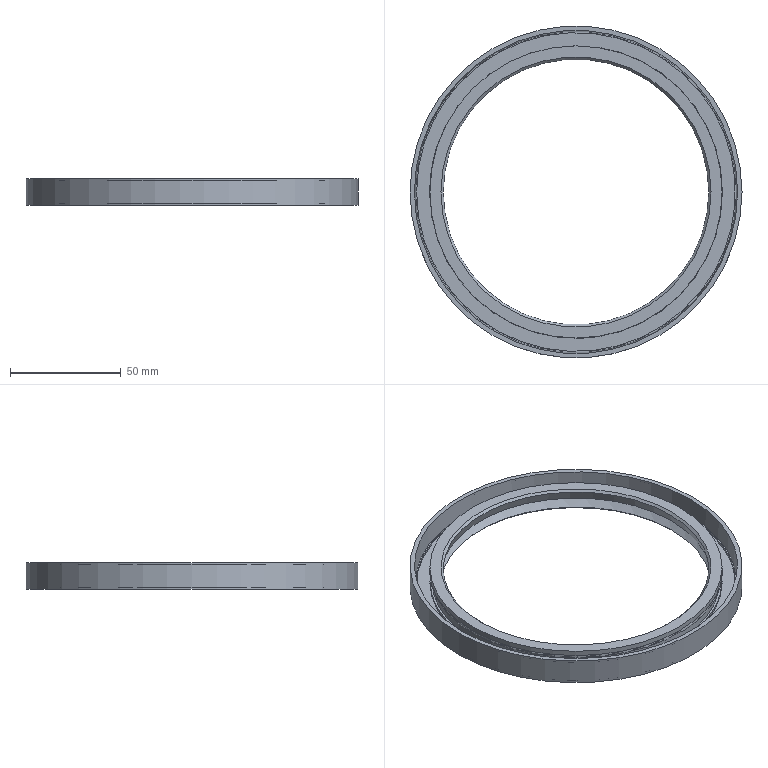Component | NX | T13871-1992_2 | 1 solid | 28 faces | volume 26333 mm3 | plane 10 | cone 9 | cylinder 7 | torus 2 | commonest cylinder face diameters 132 x2 150 x1 130 x1 149 x1 147 x1 144 x1